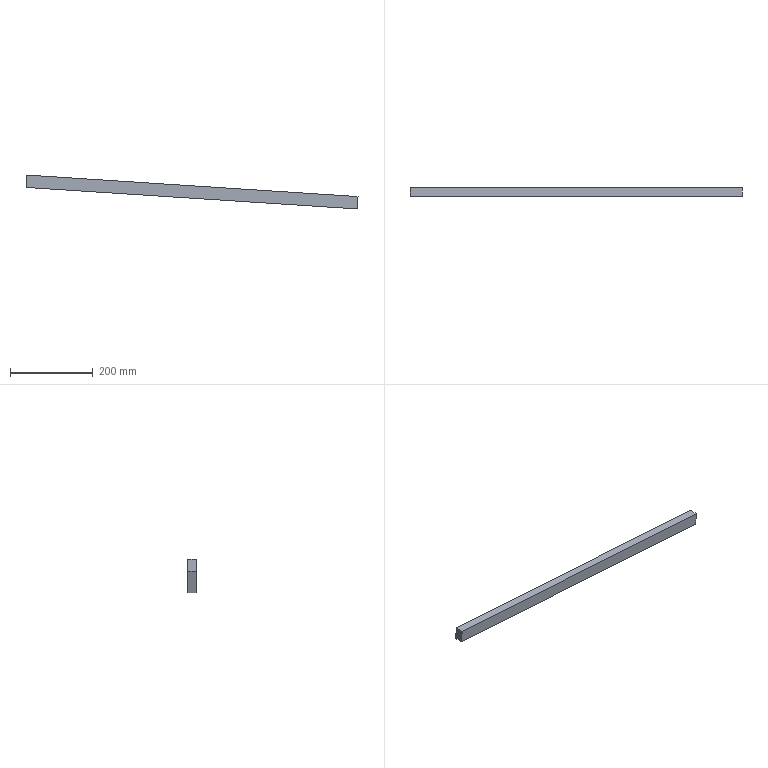Component | SolidWorks | WorkSlat-2 | 1 solid | 6 faces | box 800.26 x 20 x 81.73 mm | volume 480000 mm3 | plane 6
build123d program:
from build123d import *

# Parameters (mm, degrees)
SKETCH1_W           = 20
SKETCH1_H           = 30
BOSS_EXTRUDE1_DEPTH = 800


with BuildPart() as part:
    # Sketch1 → Boss-Extrude1 (new body)
    with BuildSketch(Plane.XY):
        with Locations((59.241, 643.295)):
            Rectangle(SKETCH1_W, SKETCH1_H)
    extrude(amount=BOSS_EXTRUDE1_DEPTH)


solid = part.part

# Placed as in the assembly
solid = solid.moved(Location((362.537, -816.759, -1033.166), (0, -86.288, -90)))
STEP:
#1=CARTESIAN_POINT('',(-15.479,-34.882,-12.774));
#2=VERTEX_POINT('',#1);
#3=CARTESIAN_POINT('',(-15.555,-34.882,-13.953));
#4=VERTEX_POINT('',#3);
#5=CARTESIAN_POINT('',(-15.555,-34.882,-13.953));
#6=DIRECTION('',(-0.06474,-0.,-0.9979));
#7=VECTOR('',#6,39.37);
#8=LINE('',#5,#7);
#9=EDGE_CURVE('',#2,#4,#8,.T.);
#10=ORIENTED_EDGE('',*,*,#9,.T.);
#11=CARTESIAN_POINT('',(15.875,-34.882,-15.992));
#12=VERTEX_POINT('',#11);
#13=CARTESIAN_POINT('',(15.875,-34.882,-15.992));
#14=DIRECTION('',(-0.9979,-0.,0.06474));
#15=VECTOR('',#14,39.37);
#16=LINE('',#13,#15);
#17=EDGE_CURVE('',#12,#4,#16,.T.);
#18=ORIENTED_EDGE('',*,*,#17,.F.);
#19=CARTESIAN_POINT('',(15.951,-34.882,-14.813));
#20=VERTEX_POINT('',#19);
#21=CARTESIAN_POINT('',(15.875,-34.882,-15.992));
#22=DIRECTION('',(-0.06474,-0.,-0.9979));
#23=VECTOR('',#22,39.37);
#24=LINE('',#21,#23);
#25=EDGE_CURVE('',#20,#12,#24,.T.);
#26=ORIENTED_EDGE('',*,*,#25,.F.);
#27=CARTESIAN_POINT('',(15.951,-34.882,-14.813));
#28=DIRECTION('',(-0.9979,-0.,0.06474));
#29=VECTOR('',#28,39.37);
#30=LINE('',#27,#29);
#31=EDGE_CURVE('',#20,#2,#30,.T.);
#32=ORIENTED_EDGE('',*,*,#31,.T.);
#33=EDGE_LOOP('',(#10,#18,#26,#32));
#34=FACE_OUTER_BOUND('',#33,.T.);
#35=CARTESIAN_POINT('',(15.875,-34.882,-15.992));
#36=DIRECTION('',(-0.,1.,0.));
#37=DIRECTION('',(0.9979,0.,-0.06474));
#38=AXIS2_PLACEMENT_3D('',#35,#36,#37);
#39=PLANE('',#38);
#40=ADVANCED_FACE('',(#34),#39,.F.);
#41=CARTESIAN_POINT('',(-15.555,-34.094,-13.953));
#42=VERTEX_POINT('',#41);
#43=CARTESIAN_POINT('',(-15.555,-34.094,-13.953));
#44=DIRECTION('',(-0.,1.,0.));
#45=VECTOR('',#44,39.37);
#46=LINE('',#43,#45);
#47=EDGE_CURVE('',#4,#42,#46,.T.);
#48=ORIENTED_EDGE('',*,*,#47,.T.);
#49=CARTESIAN_POINT('',(15.875,-34.094,-15.992));
#50=VERTEX_POINT('',#49);
#51=CARTESIAN_POINT('',(15.875,-34.094,-15.992));
#52=DIRECTION('',(-0.9979,-0.,0.06474));
#53=VECTOR('',#52,39.37);
#54=LINE('',#51,#53);
#55=EDGE_CURVE('',#50,#42,#54,.T.);
#56=ORIENTED_EDGE('',*,*,#55,.F.);
#57=CARTESIAN_POINT('',(15.875,-34.094,-15.992));
#58=DIRECTION('',(-0.,1.,0.));
#59=VECTOR('',#58,39.37);
#60=LINE('',#57,#59);
#61=EDGE_CURVE('',#12,#50,#60,.T.);
#62=ORIENTED_EDGE('',*,*,#61,.F.);
#63=ORIENTED_EDGE('',*,*,#17,.T.);
#64=EDGE_LOOP('',(#48,#56,#62,#63));
#65=FACE_OUTER_BOUND('',#64,.T.);
#66=CARTESIAN_POINT('',(15.875,-34.094,-15.992));
#67=DIRECTION('',(0.06474,0.,0.9979));
#68=DIRECTION('',(-0.9979,-0.,0.06474));
#69=AXIS2_PLACEMENT_3D('',#66,#67,#68);
#70=PLANE('',#69);
#71=ADVANCED_FACE('',(#65),#70,.F.);
#72=CARTESIAN_POINT('',(-15.479,-34.094,-12.774));
#73=VERTEX_POINT('',#72);
#74=CARTESIAN_POINT('',(-15.555,-34.094,-13.953));
#75=DIRECTION('',(0.06474,-0.,0.9979));
#76=VECTOR('',#75,39.37);
#77=LINE('',#74,#76);
#78=EDGE_CURVE('',#42,#73,#77,.T.);
#79=ORIENTED_EDGE('',*,*,#78,.T.);
#80=CARTESIAN_POINT('',(15.951,-34.094,-14.813));
#81=VERTEX_POINT('',#80);
#82=CARTESIAN_POINT('',(15.951,-34.094,-14.813));
#83=DIRECTION('',(-0.9979,-0.,0.06474));
#84=VECTOR('',#83,39.37);
#85=LINE('',#82,#84);
#86=EDGE_CURVE('',#81,#73,#85,.T.);
#87=ORIENTED_EDGE('',*,*,#86,.F.);
#88=CARTESIAN_POINT('',(15.875,-34.094,-15.992));
#89=DIRECTION('',(0.06474,-0.,0.9979));
#90=VECTOR('',#89,39.37);
#91=LINE('',#88,#90);
#92=EDGE_CURVE('',#50,#81,#91,.T.);
#93=ORIENTED_EDGE('',*,*,#92,.F.);
#94=ORIENTED_EDGE('',*,*,#55,.T.);
#95=EDGE_LOOP('',(#79,#87,#93,#94));
#96=FACE_OUTER_BOUND('',#95,.T.);
#97=CARTESIAN_POINT('',(15.875,-34.094,-15.992));
#98=DIRECTION('',(0.,-1.,-0.));
#99=DIRECTION('',(-0.06474,0.,-0.9979));
#100=AXIS2_PLACEMENT_3D('',#97,#98,#99);
#101=PLANE('',#100);
#102=ADVANCED_FACE('',(#96),#101,.F.);
#103=CARTESIAN_POINT('',(-15.479,-34.094,-12.774));
#104=DIRECTION('',(0.,-1.,-0.));
#105=VECTOR('',#104,39.37);
#106=LINE('',#103,#105);
#107=EDGE_CURVE('',#73,#2,#106,.T.);
#108=ORIENTED_EDGE('',*,*,#107,.T.);
#109=ORIENTED_EDGE('',*,*,#31,.F.);
#110=CARTESIAN_POINT('',(15.951,-34.094,-14.813));
#111=DIRECTION('',(0.,-1.,-0.));
#112=VECTOR('',#111,39.37);
#113=LINE('',#110,#112);
#114=EDGE_CURVE('',#81,#20,#113,.T.);
#115=ORIENTED_EDGE('',*,*,#114,.F.);
#116=ORIENTED_EDGE('',*,*,#86,.T.);
#117=EDGE_LOOP('',(#108,#109,#115,#116));
#118=FACE_OUTER_BOUND('',#117,.T.);
#119=CARTESIAN_POINT('',(15.951,-34.094,-14.813));
#120=DIRECTION('',(-0.06474,-0.,-0.9979));
#121=DIRECTION('',(0.9979,0.,-0.06474));
#122=AXIS2_PLACEMENT_3D('',#119,#120,#121);
#123=PLANE('',#122);
#124=ADVANCED_FACE('',(#118),#123,.F.);
#125=ORIENTED_EDGE('',*,*,#25,.T.);
#126=ORIENTED_EDGE('',*,*,#61,.T.);
#127=ORIENTED_EDGE('',*,*,#92,.T.);
#128=ORIENTED_EDGE('',*,*,#114,.T.);
#129=EDGE_LOOP('',(#125,#126,#127,#128));
#130=FACE_OUTER_BOUND('',#129,.T.);
#131=CARTESIAN_POINT('',(17.552,-32.156,9.871));
#132=DIRECTION('',(0.9979,0.,-0.06474));
#133=DIRECTION('',(0.,-1.,-0.));
#134=AXIS2_PLACEMENT_3D('',#131,#132,#133);
#135=PLANE('',#134);
#136=ADVANCED_FACE('',(#130),#135,.T.);
#137=ORIENTED_EDGE('',*,*,#9,.F.);
#138=ORIENTED_EDGE('',*,*,#107,.F.);
#139=ORIENTED_EDGE('',*,*,#78,.F.);
#140=ORIENTED_EDGE('',*,*,#47,.F.);
#141=EDGE_LOOP('',(#137,#138,#139,#140));
#142=FACE_OUTER_BOUND('',#141,.T.);
#143=CARTESIAN_POINT('',(-13.878,-32.156,11.91));
#144=DIRECTION('',(0.9979,0.,-0.06474));
#145=DIRECTION('',(0.,-1.,-0.));
#146=AXIS2_PLACEMENT_3D('',#143,#144,#145);
#147=PLANE('',#146);
#148=ADVANCED_FACE('',(#142),#147,.F.);
#149=CLOSED_SHELL('',(#40,#71,#102,#124,#136,#148));
#150=MANIFOLD_SOLID_BREP('',#149);
#151=CARTESIAN_POINT('',(0.,0.,0.));
#152=DIRECTION('',(0.,0.,1.));
#153=DIRECTION('',(1.,0.,0.));
#154=AXIS2_PLACEMENT_3D('',#151,#152,#153);
#155=(LENGTH_UNIT()NAMED_UNIT(*)SI_UNIT($,.METRE.));
#156=LENGTH_MEASURE_WITH_UNIT(LENGTH_MEASURE(0.0254),#155);
#157=DIMENSIONAL_EXPONENTS(1.,0.,0.,0.,0.,0.,0.);
#158=(CONVERSION_BASED_UNIT('',#156)LENGTH_UNIT()NAMED_UNIT(#157));
#159=UNCERTAINTY_MEASURE_WITH_UNIT(LENGTH_MEASURE(0.00001),#158,'','');
#160=(NAMED_UNIT(*)PLANE_ANGLE_UNIT()SI_UNIT($,.RADIAN.));
#161=(NAMED_UNIT(*)SI_UNIT($,.STERADIAN.)SOLID_ANGLE_UNIT());
#162=(GEOMETRIC_REPRESENTATION_CONTEXT(3)GLOBAL_UNCERTAINTY_ASSIGNED_CONTEXT((#159))GLOBAL_UNIT_ASSIGNED_CONTEXT((#158,#160,#161))REPRESENTATION_CONTEXT('',''));
#163=ADVANCED_BREP_SHAPE_REPRESENTATION('',(#150,#154),#162);
#164=COLOUR_RGB('',0.7922,0.8196,0.9333);
#165=FILL_AREA_STYLE_COLOUR('',#164);
#166=FILL_AREA_STYLE('',(#165));
#167=SURFACE_STYLE_FILL_AREA(#166);
#168=SURFACE_SIDE_STYLE('',(#167));
#169=SURFACE_STYLE_USAGE(.BOTH.,#168);
#170=PRESENTATION_STYLE_ASSIGNMENT((#169));
#171=STYLED_ITEM('',(#170),#150);
#172=(LENGTH_UNIT()NAMED_UNIT(*)SI_UNIT($,.METRE.));
#173=LENGTH_MEASURE_WITH_UNIT(LENGTH_MEASURE(0.0254),#172);
#174=DIMENSIONAL_EXPONENTS(1.,0.,0.,0.,0.,0.,0.);
#175=(CONVERSION_BASED_UNIT('',#173)LENGTH_UNIT()NAMED_UNIT(#174));
#176=UNCERTAINTY_MEASURE_WITH_UNIT(LENGTH_MEASURE(0.00001),#175,'','');
#177=(NAMED_UNIT(*)PLANE_ANGLE_UNIT()SI_UNIT($,.RADIAN.));
#178=(NAMED_UNIT(*)SI_UNIT($,.STERADIAN.)SOLID_ANGLE_UNIT());
#179=(GEOMETRIC_REPRESENTATION_CONTEXT(3)GLOBAL_UNCERTAINTY_ASSIGNED_CONTEXT((#176))GLOBAL_UNIT_ASSIGNED_CONTEXT((#175,#177,#178))REPRESENTATION_CONTEXT('',''));
#180=MECHANICAL_DESIGN_GEOMETRIC_PRESENTATION_REPRESENTATION('',(#171),#179);
#181=PRESENTATION_LAYER_ASSIGNMENT('','',(#171));